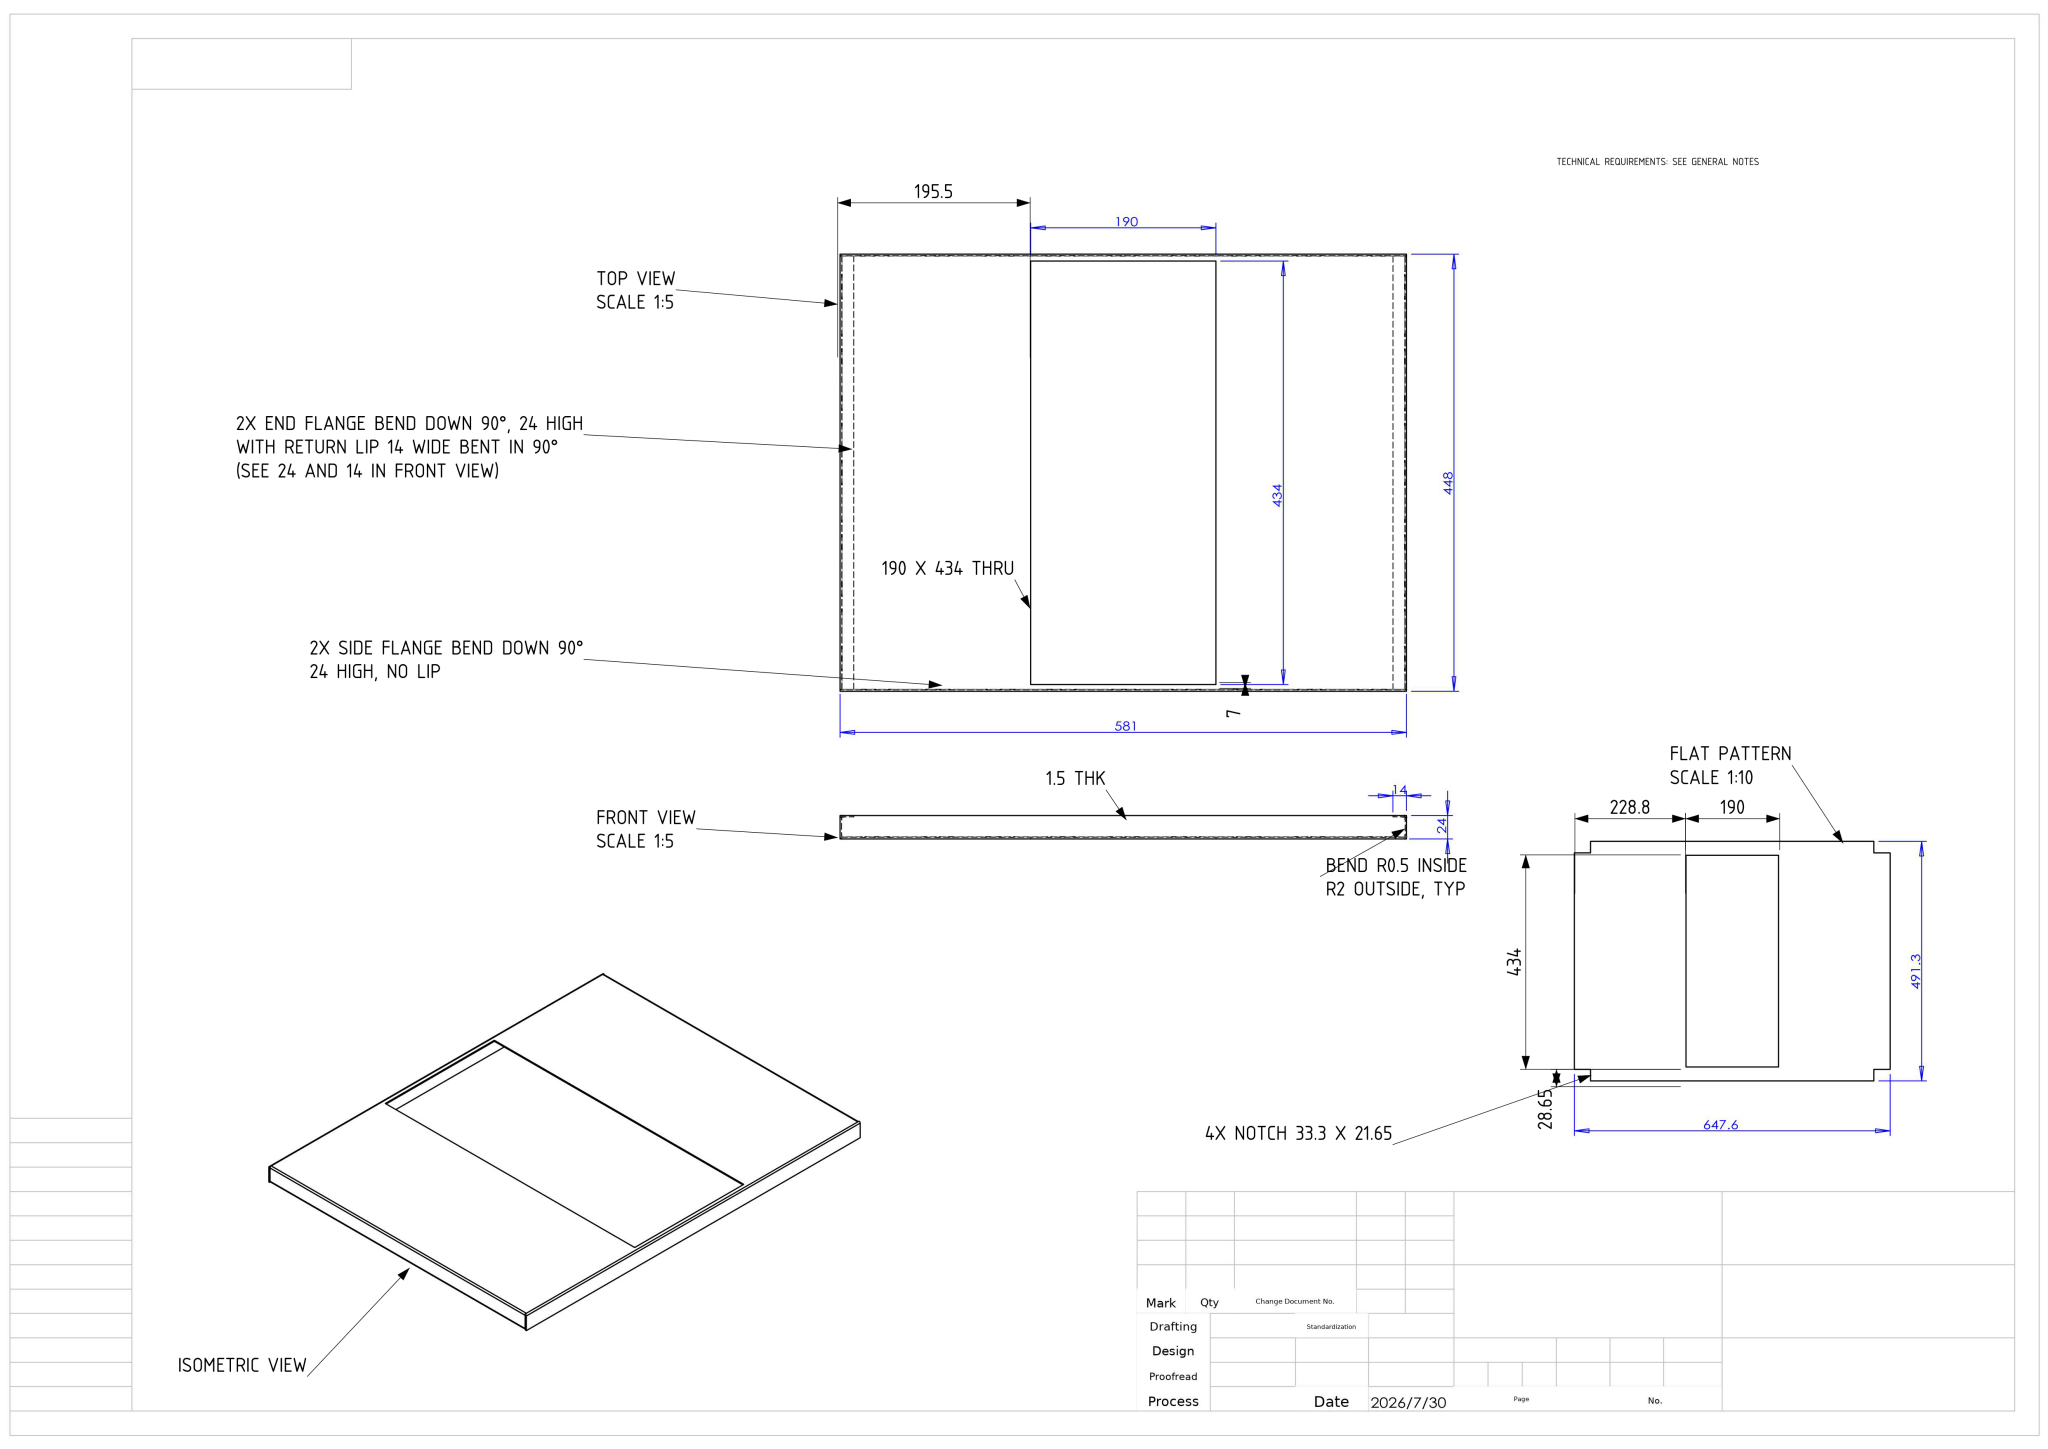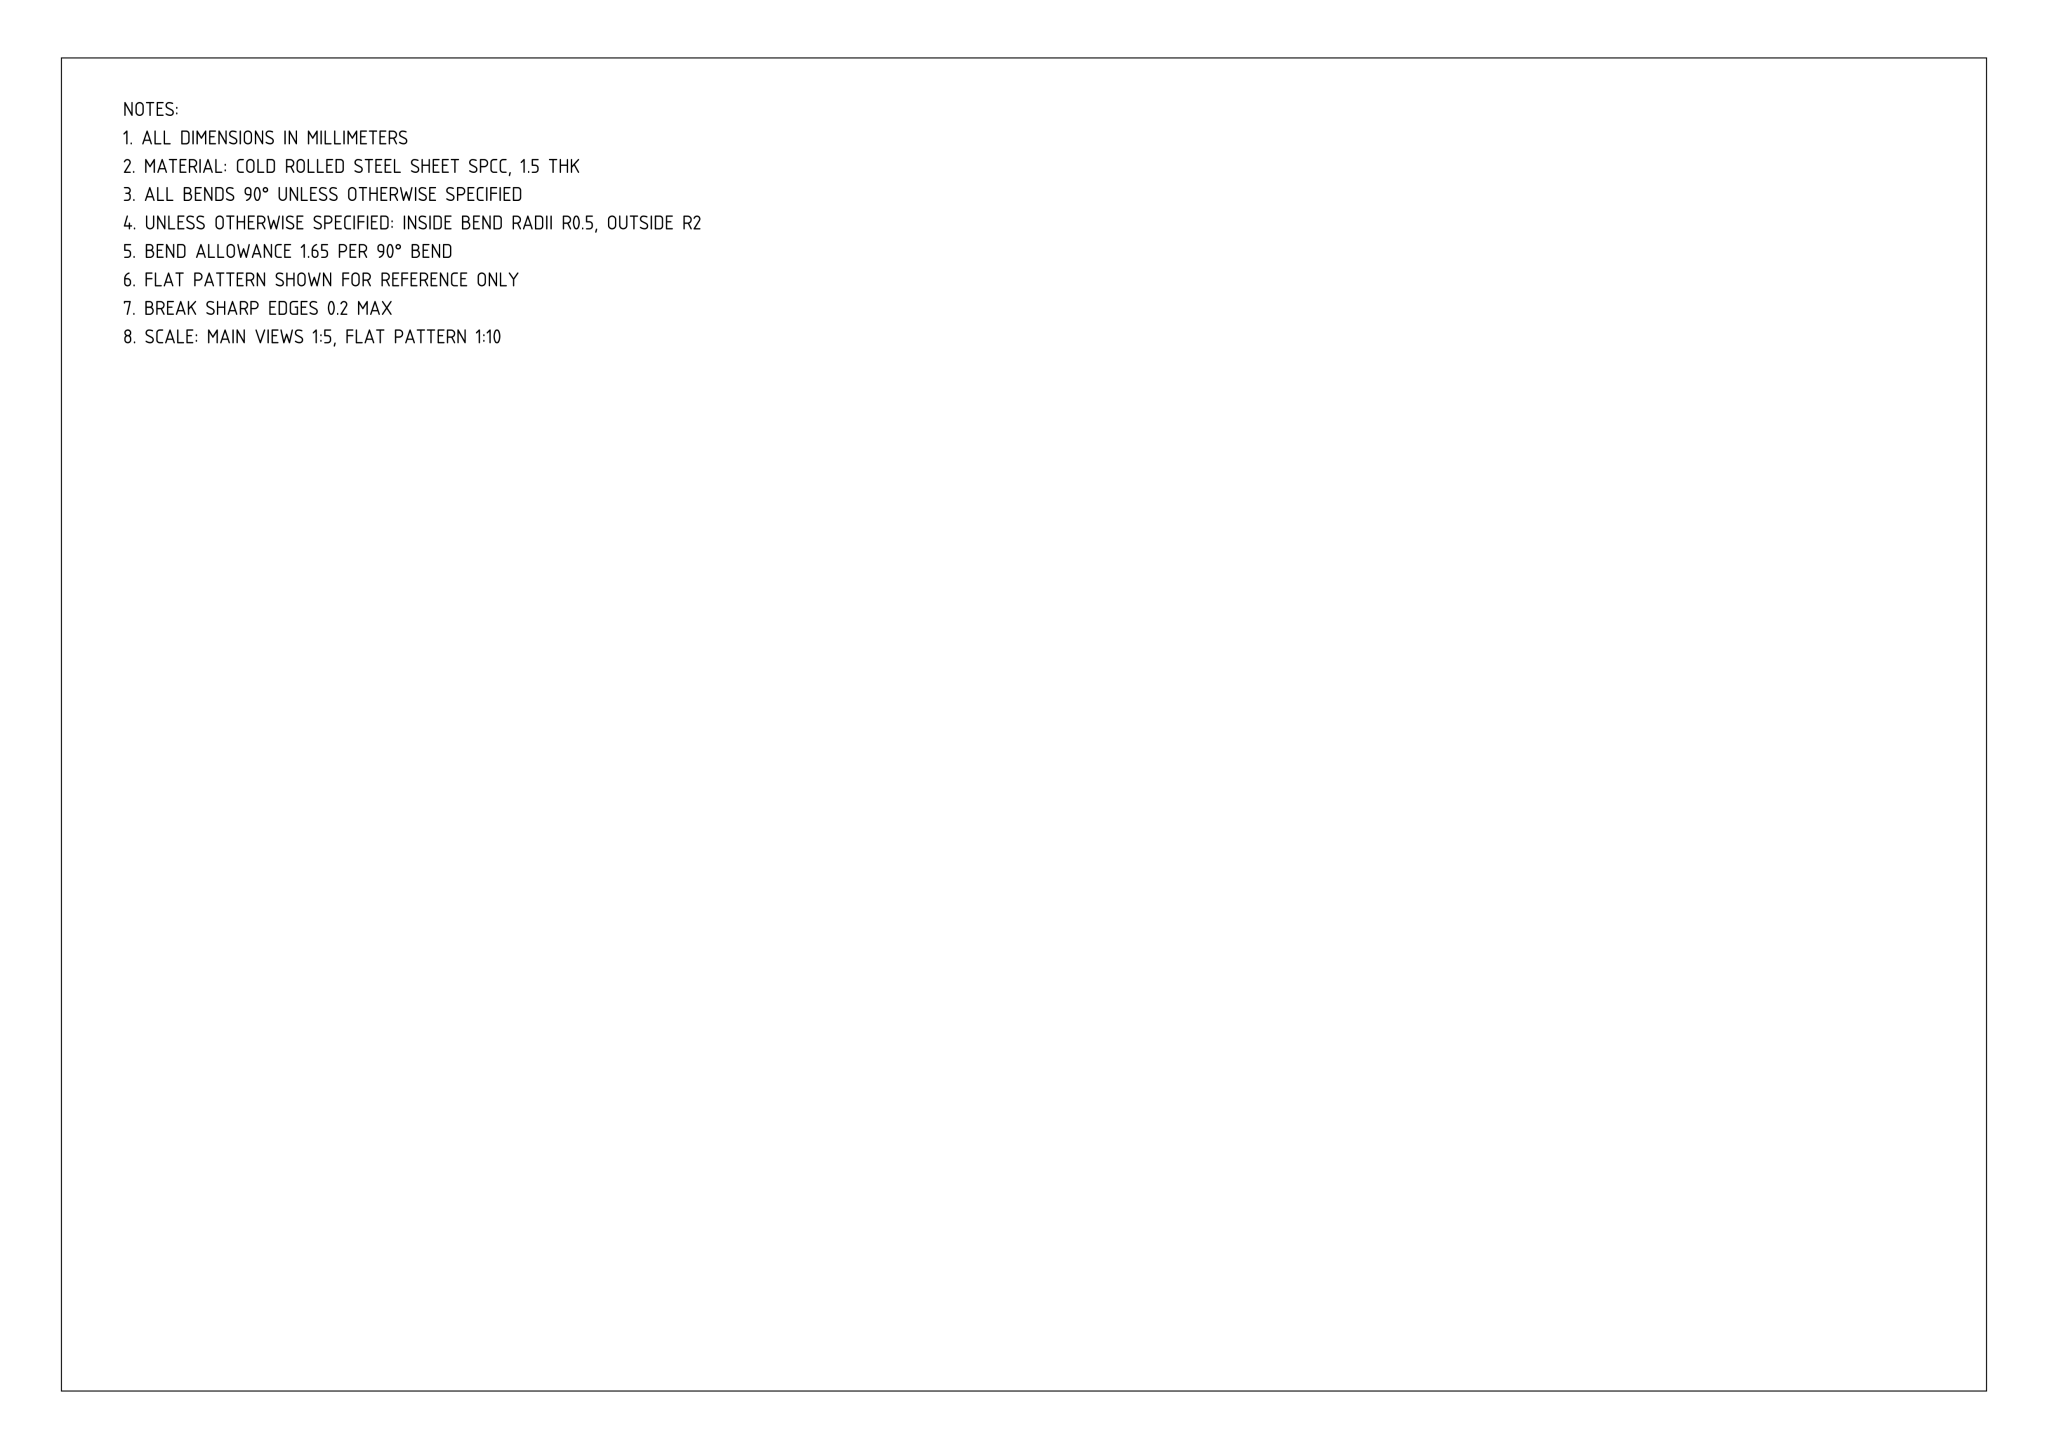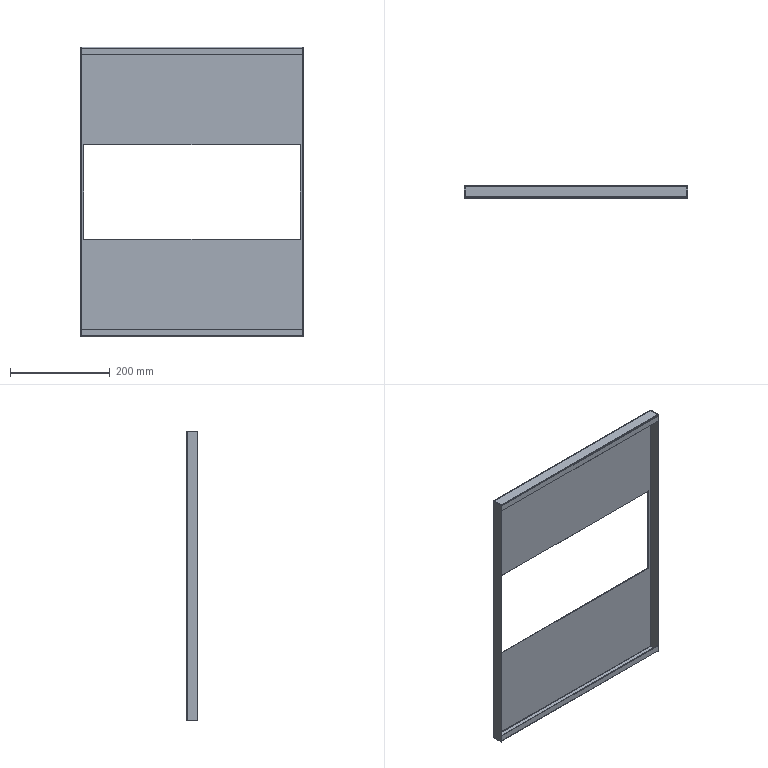Part | NX | mm | 1 solid | 62 faces | box 448 x 24 x 581 mm | volume 350215 mm3 | plane 50 | cylinder 12 | commonest cylinder face diameters 4 x6 1 x6